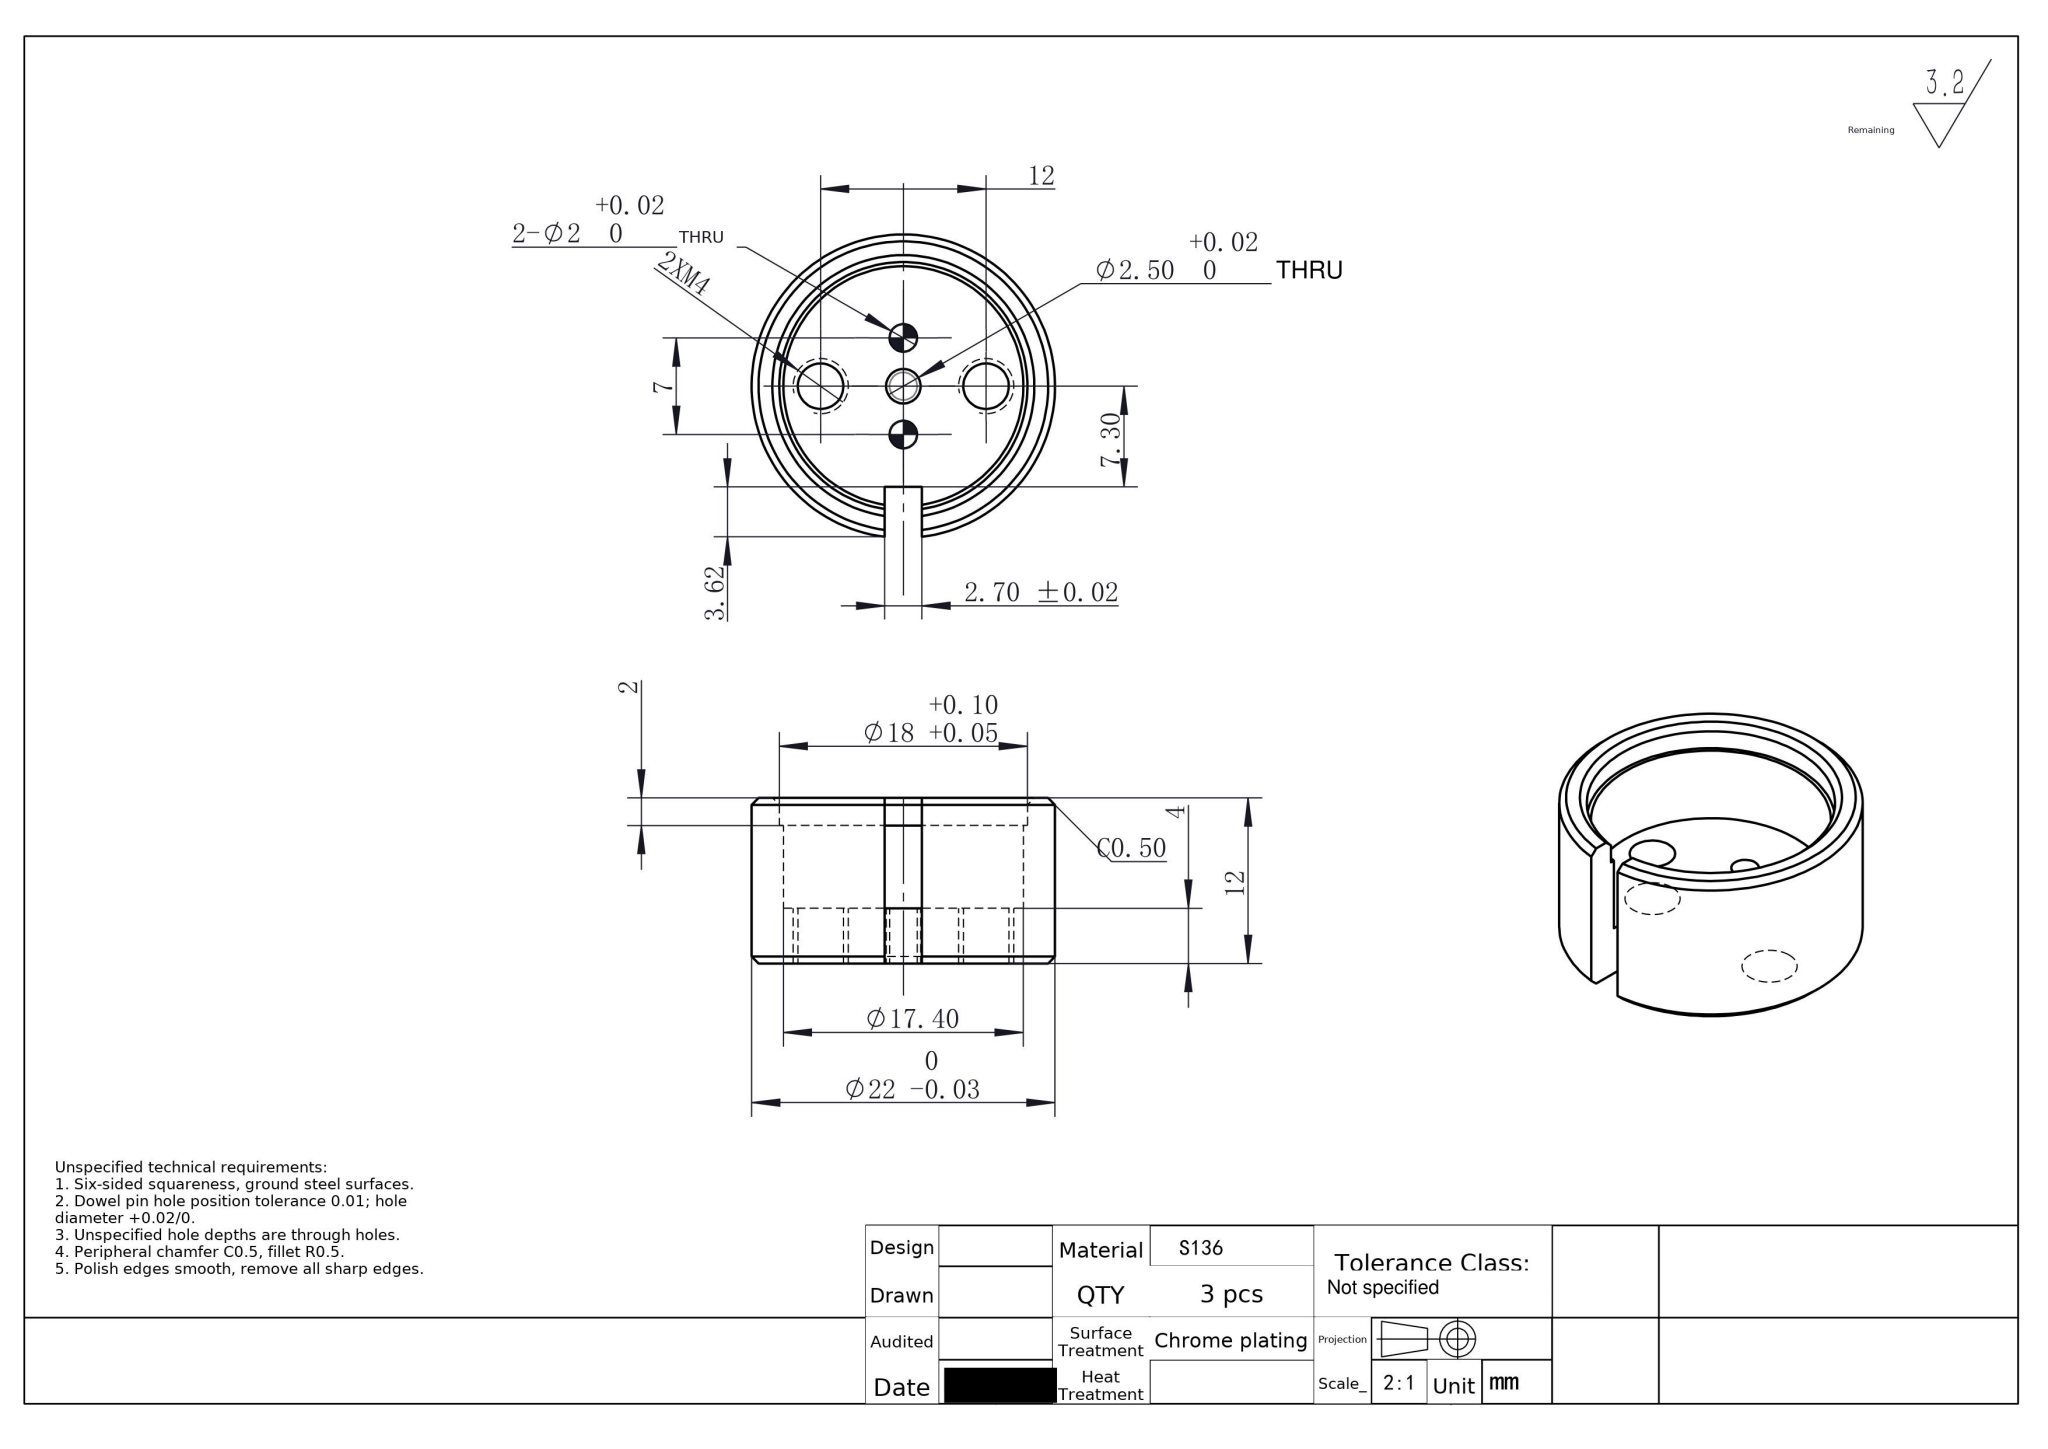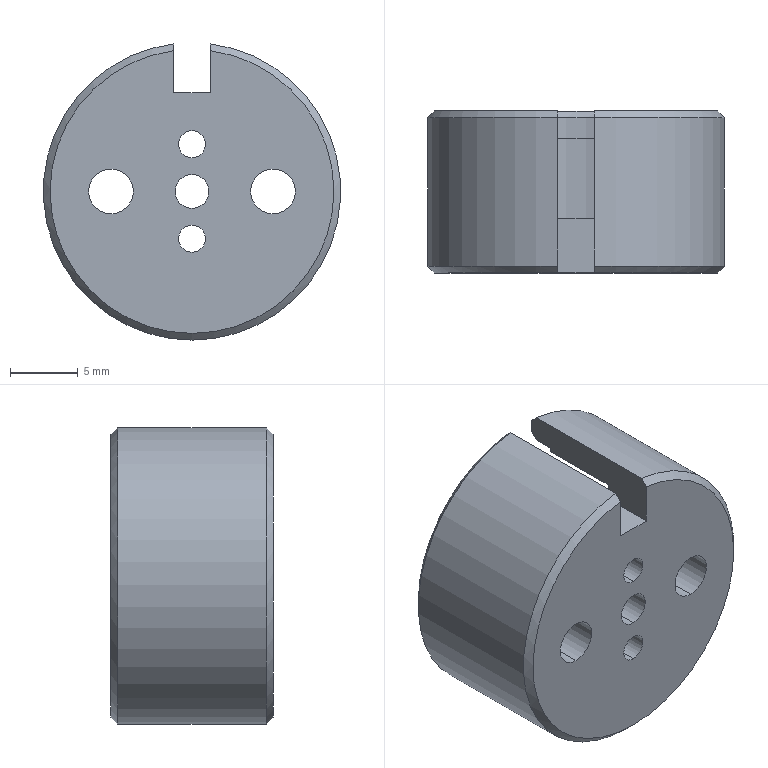Part | NX | mm | 1 solid | 25 faces | box 22 x 12 x 21.92 mm | volume 2402 mm3 | cylinder 14 | plane 7 | cone 4 | commonest cylinder face diameters 2 x4 3.3 x4 22 x2 2.5 x2 18 x1 17.4 x1
STEP:
#1=CARTESIAN_POINT('',(0.,0.,-4.5));
#2=VERTEX_POINT('',#1);
#3=CARTESIAN_POINT('',(0.,0.,-2.5));
#4=VERTEX_POINT('',#3);
#5=CARTESIAN_POINT('',(0.,0.,-3.5));
#6=DIRECTION('',(0.,1.,0.));
#7=DIRECTION('',(0.,0.,1.));
#8=AXIS2_PLACEMENT_3D('',#5,#6,#7);
#9=CIRCLE('',#8,1.);
#10=EDGE_CURVE('',#2,#4,#9,.T.);
#11=ORIENTED_EDGE('',*,*,#10,.F.);
#12=CARTESIAN_POINT('',(0.,4.,-4.5));
#13=VERTEX_POINT('',#12);
#14=CARTESIAN_POINT('',(0.,4.,-4.5));
#15=DIRECTION('',(0.,1.,0.));
#16=VECTOR('',#15,1000.);
#17=LINE('',#14,#16);
#18=EDGE_CURVE('',#2,#13,#17,.T.);
#19=ORIENTED_EDGE('',*,*,#18,.T.);
#20=CARTESIAN_POINT('',(0.,4.,-2.5));
#21=VERTEX_POINT('',#20);
#22=CARTESIAN_POINT('',(0.,4.,-3.5));
#23=DIRECTION('',(0.,1.,0.));
#24=DIRECTION('',(0.,0.,1.));
#25=AXIS2_PLACEMENT_3D('',#22,#23,#24);
#26=CIRCLE('',#25,1.);
#27=EDGE_CURVE('',#13,#21,#26,.T.);
#28=ORIENTED_EDGE('',*,*,#27,.T.);
#29=CARTESIAN_POINT('',(0.,4.,-2.5));
#30=DIRECTION('',(0.,1.,0.));
#31=VECTOR('',#30,1000.);
#32=LINE('',#29,#31);
#33=EDGE_CURVE('',#4,#21,#32,.T.);
#34=ORIENTED_EDGE('',*,*,#33,.F.);
#35=EDGE_LOOP('',(#11,#19,#28,#34));
#36=FACE_OUTER_BOUND('',#35,.T.);
#37=CARTESIAN_POINT('',(0.,4.,-3.5));
#38=DIRECTION('',(0.,1.,0.));
#39=DIRECTION('',(0.,0.,1.));
#40=AXIS2_PLACEMENT_3D('',#37,#38,#39);
#41=CYLINDRICAL_SURFACE('',#40,1.);
#42=ADVANCED_FACE('',(#36),#41,.F.);
#43=CARTESIAN_POINT('',(0.,0.,2.5));
#44=VERTEX_POINT('',#43);
#45=CARTESIAN_POINT('',(0.,0.,4.5));
#46=VERTEX_POINT('',#45);
#47=CARTESIAN_POINT('',(0.,0.,3.5));
#48=DIRECTION('',(0.,1.,0.));
#49=DIRECTION('',(0.,0.,1.));
#50=AXIS2_PLACEMENT_3D('',#47,#48,#49);
#51=CIRCLE('',#50,1.);
#52=EDGE_CURVE('',#44,#46,#51,.T.);
#53=ORIENTED_EDGE('',*,*,#52,.F.);
#54=CARTESIAN_POINT('',(0.,4.,2.5));
#55=VERTEX_POINT('',#54);
#56=CARTESIAN_POINT('',(0.,4.,2.5));
#57=DIRECTION('',(0.,1.,0.));
#58=VECTOR('',#57,1000.);
#59=LINE('',#56,#58);
#60=EDGE_CURVE('',#44,#55,#59,.T.);
#61=ORIENTED_EDGE('',*,*,#60,.T.);
#62=CARTESIAN_POINT('',(0.,4.,4.5));
#63=VERTEX_POINT('',#62);
#64=CARTESIAN_POINT('',(0.,4.,3.5));
#65=DIRECTION('',(0.,1.,0.));
#66=DIRECTION('',(0.,0.,1.));
#67=AXIS2_PLACEMENT_3D('',#64,#65,#66);
#68=CIRCLE('',#67,1.);
#69=EDGE_CURVE('',#55,#63,#68,.T.);
#70=ORIENTED_EDGE('',*,*,#69,.T.);
#71=CARTESIAN_POINT('',(0.,4.,4.5));
#72=DIRECTION('',(0.,1.,0.));
#73=VECTOR('',#72,1000.);
#74=LINE('',#71,#73);
#75=EDGE_CURVE('',#46,#63,#74,.T.);
#76=ORIENTED_EDGE('',*,*,#75,.F.);
#77=EDGE_LOOP('',(#53,#61,#70,#76));
#78=FACE_OUTER_BOUND('',#77,.T.);
#79=CARTESIAN_POINT('',(0.,4.,3.5));
#80=DIRECTION('',(0.,1.,0.));
#81=DIRECTION('',(0.,0.,1.));
#82=AXIS2_PLACEMENT_3D('',#79,#80,#81);
#83=CYLINDRICAL_SURFACE('',#82,1.);
#84=ADVANCED_FACE('',(#78),#83,.F.);
#85=CARTESIAN_POINT('',(0.,12.,-10.5));
#86=VERTEX_POINT('',#85);
#87=CARTESIAN_POINT('',(-1.35,12.,10.413));
#88=VERTEX_POINT('',#87);
#89=CARTESIAN_POINT('',(0.,12.,0.));
#90=DIRECTION('',(0.,1.,0.));
#91=DIRECTION('',(0.,0.,1.));
#92=AXIS2_PLACEMENT_3D('',#89,#90,#91);
#93=CIRCLE('',#92,10.5);
#94=EDGE_CURVE('',#86,#88,#93,.T.);
#95=ORIENTED_EDGE('',*,*,#94,.F.);
#96=CARTESIAN_POINT('',(0.,11.5,-11.));
#97=VERTEX_POINT('',#96);
#98=CARTESIAN_POINT('',(0.,12.,-10.5));
#99=DIRECTION('',(0.,-0.7071,-0.7071));
#100=VECTOR('',#99,1000.);
#101=LINE('',#98,#100);
#102=EDGE_CURVE('',#86,#97,#101,.T.);
#103=ORIENTED_EDGE('',*,*,#102,.T.);
#104=CARTESIAN_POINT('',(-1.35,11.5,10.917));
#105=VERTEX_POINT('',#104);
#106=CARTESIAN_POINT('',(0.,11.5,0.));
#107=DIRECTION('',(0.,-1.,0.));
#108=DIRECTION('',(0.,0.,1.));
#109=AXIS2_PLACEMENT_3D('',#106,#107,#108);
#110=CIRCLE('',#109,11.);
#111=EDGE_CURVE('',#105,#97,#110,.T.);
#112=ORIENTED_EDGE('',*,*,#111,.F.);
#113=CARTESIAN_POINT('',(-1.35,12.,10.413));
#114=CARTESIAN_POINT('',(-1.35,11.833,10.581));
#115=CARTESIAN_POINT('',(-1.35,11.667,10.749));
#116=CARTESIAN_POINT('',(-1.35,11.5,10.917));
#117=B_SPLINE_CURVE_WITH_KNOTS('',3,(#113,#114,#115,#116),.UNSPECIFIED.,.F.,.F.,(4,4),(0.006562,0.007272),.UNSPECIFIED.);
#118=EDGE_CURVE('',#88,#105,#117,.T.);
#119=ORIENTED_EDGE('',*,*,#118,.F.);
#120=EDGE_LOOP('',(#95,#103,#112,#119));
#121=FACE_OUTER_BOUND('',#120,.T.);
#122=CARTESIAN_POINT('',(0.,12.,0.));
#123=DIRECTION('',(0.,-1.,0.));
#124=DIRECTION('',(0.,0.,-1.));
#125=AXIS2_PLACEMENT_3D('',#122,#123,#124);
#126=CONICAL_SURFACE('',#125,10.5,0.7854);
#127=ADVANCED_FACE('',(#121),#126,.T.);
#128=ORIENTED_EDGE('',*,*,#111,.T.);
#129=CARTESIAN_POINT('',(0.,0.5,-11.));
#130=VERTEX_POINT('',#129);
#131=CARTESIAN_POINT('',(0.,12.,-11.));
#132=DIRECTION('',(0.,-1.,0.));
#133=VECTOR('',#132,1000.);
#134=LINE('',#131,#133);
#135=EDGE_CURVE('',#97,#130,#134,.T.);
#136=ORIENTED_EDGE('',*,*,#135,.T.);
#137=CARTESIAN_POINT('',(-1.35,0.5,10.917));
#138=VERTEX_POINT('',#137);
#139=CARTESIAN_POINT('',(0.,0.5,0.));
#140=DIRECTION('',(0.,1.,0.));
#141=DIRECTION('',(0.,0.,1.));
#142=AXIS2_PLACEMENT_3D('',#139,#140,#141);
#143=CIRCLE('',#142,11.);
#144=EDGE_CURVE('',#130,#138,#143,.T.);
#145=ORIENTED_EDGE('',*,*,#144,.T.);
#146=CARTESIAN_POINT('',(-1.35,12.,10.917));
#147=DIRECTION('',(0.,1.,0.));
#148=VECTOR('',#147,1000.);
#149=LINE('',#146,#148);
#150=EDGE_CURVE('',#138,#105,#149,.T.);
#151=ORIENTED_EDGE('',*,*,#150,.T.);
#152=EDGE_LOOP('',(#128,#136,#145,#151));
#153=FACE_OUTER_BOUND('',#152,.T.);
#154=CARTESIAN_POINT('',(0.,12.,0.));
#155=DIRECTION('',(0.,-1.,0.));
#156=DIRECTION('',(0.,0.,-1.));
#157=AXIS2_PLACEMENT_3D('',#154,#155,#156);
#158=CYLINDRICAL_SURFACE('',#157,11.);
#159=ADVANCED_FACE('',(#153),#158,.T.);
#160=CARTESIAN_POINT('',(0.,0.,-1.25));
#161=VERTEX_POINT('',#160);
#162=CARTESIAN_POINT('',(0.,0.,1.25));
#163=VERTEX_POINT('',#162);
#164=CARTESIAN_POINT('',(0.,0.,0.));
#165=DIRECTION('',(0.,1.,0.));
#166=DIRECTION('',(0.,0.,1.));
#167=AXIS2_PLACEMENT_3D('',#164,#165,#166);
#168=CIRCLE('',#167,1.25);
#169=EDGE_CURVE('',#161,#163,#168,.T.);
#170=ORIENTED_EDGE('',*,*,#169,.F.);
#171=CARTESIAN_POINT('',(0.,4.,-1.25));
#172=VERTEX_POINT('',#171);
#173=CARTESIAN_POINT('',(0.,0.,-1.25));
#174=DIRECTION('',(0.,1.,0.));
#175=VECTOR('',#174,1000.);
#176=LINE('',#173,#175);
#177=EDGE_CURVE('',#161,#172,#176,.T.);
#178=ORIENTED_EDGE('',*,*,#177,.T.);
#179=CARTESIAN_POINT('',(0.,4.,1.25));
#180=VERTEX_POINT('',#179);
#181=CARTESIAN_POINT('',(0.,4.,0.));
#182=DIRECTION('',(0.,-1.,0.));
#183=DIRECTION('',(0.,0.,1.));
#184=AXIS2_PLACEMENT_3D('',#181,#182,#183);
#185=CIRCLE('',#184,1.25);
#186=EDGE_CURVE('',#180,#172,#185,.T.);
#187=ORIENTED_EDGE('',*,*,#186,.F.);
#188=CARTESIAN_POINT('',(0.,0.,1.25));
#189=DIRECTION('',(0.,1.,0.));
#190=VECTOR('',#189,1000.);
#191=LINE('',#188,#190);
#192=EDGE_CURVE('',#163,#180,#191,.T.);
#193=ORIENTED_EDGE('',*,*,#192,.F.);
#194=EDGE_LOOP('',(#170,#178,#187,#193));
#195=FACE_OUTER_BOUND('',#194,.T.);
#196=CARTESIAN_POINT('',(0.,0.,0.));
#197=DIRECTION('',(0.,1.,0.));
#198=DIRECTION('',(0.,0.,1.));
#199=AXIS2_PLACEMENT_3D('',#196,#197,#198);
#200=CYLINDRICAL_SURFACE('',#199,1.25);
#201=ADVANCED_FACE('',(#195),#200,.F.);
#202=CARTESIAN_POINT('',(-6.,4.,1.65));
#203=VERTEX_POINT('',#202);
#204=CARTESIAN_POINT('',(-6.,4.,-1.65));
#205=VERTEX_POINT('',#204);
#206=CARTESIAN_POINT('',(-6.,4.,0.));
#207=DIRECTION('',(0.,-1.,0.));
#208=DIRECTION('',(0.,0.,1.));
#209=AXIS2_PLACEMENT_3D('',#206,#207,#208);
#210=CIRCLE('',#209,1.65);
#211=EDGE_CURVE('',#203,#205,#210,.T.);
#212=ORIENTED_EDGE('',*,*,#211,.F.);
#213=CARTESIAN_POINT('',(-6.,-0.,1.65));
#214=VERTEX_POINT('',#213);
#215=CARTESIAN_POINT('',(-6.,0.,1.65));
#216=DIRECTION('',(0.,-1.,0.));
#217=VECTOR('',#216,1000.);
#218=LINE('',#215,#217);
#219=EDGE_CURVE('',#203,#214,#218,.T.);
#220=ORIENTED_EDGE('',*,*,#219,.T.);
#221=CARTESIAN_POINT('',(-6.,-0.,-1.65));
#222=VERTEX_POINT('',#221);
#223=CARTESIAN_POINT('',(-6.,-0.,0.));
#224=DIRECTION('',(0.,-1.,0.));
#225=DIRECTION('',(0.,0.,-1.));
#226=AXIS2_PLACEMENT_3D('',#223,#224,#225);
#227=CIRCLE('',#226,1.65);
#228=EDGE_CURVE('',#214,#222,#227,.T.);
#229=ORIENTED_EDGE('',*,*,#228,.T.);
#230=CARTESIAN_POINT('',(-6.,0.,-1.65));
#231=DIRECTION('',(0.,-1.,0.));
#232=VECTOR('',#231,1000.);
#233=LINE('',#230,#232);
#234=EDGE_CURVE('',#205,#222,#233,.T.);
#235=ORIENTED_EDGE('',*,*,#234,.F.);
#236=EDGE_LOOP('',(#212,#220,#229,#235));
#237=FACE_OUTER_BOUND('',#236,.T.);
#238=CARTESIAN_POINT('',(-6.,0.,0.));
#239=DIRECTION('',(0.,-1.,0.));
#240=DIRECTION('',(0.,0.,-1.));
#241=AXIS2_PLACEMENT_3D('',#238,#239,#240);
#242=CYLINDRICAL_SURFACE('',#241,1.65);
#243=ADVANCED_FACE('',(#237),#242,.F.);
#244=CARTESIAN_POINT('',(6.,4.,1.65));
#245=VERTEX_POINT('',#244);
#246=CARTESIAN_POINT('',(6.,4.,-1.65));
#247=VERTEX_POINT('',#246);
#248=CARTESIAN_POINT('',(6.,4.,0.));
#249=DIRECTION('',(0.,-1.,0.));
#250=DIRECTION('',(0.,0.,1.));
#251=AXIS2_PLACEMENT_3D('',#248,#249,#250);
#252=CIRCLE('',#251,1.65);
#253=EDGE_CURVE('',#245,#247,#252,.T.);
#254=ORIENTED_EDGE('',*,*,#253,.F.);
#255=CARTESIAN_POINT('',(6.,-0.,1.65));
#256=VERTEX_POINT('',#255);
#257=CARTESIAN_POINT('',(6.,0.,1.65));
#258=DIRECTION('',(0.,-1.,0.));
#259=VECTOR('',#258,1000.);
#260=LINE('',#257,#259);
#261=EDGE_CURVE('',#245,#256,#260,.T.);
#262=ORIENTED_EDGE('',*,*,#261,.T.);
#263=CARTESIAN_POINT('',(6.,-0.,-1.65));
#264=VERTEX_POINT('',#263);
#265=CARTESIAN_POINT('',(6.,-0.,0.));
#266=DIRECTION('',(0.,-1.,0.));
#267=DIRECTION('',(0.,0.,-1.));
#268=AXIS2_PLACEMENT_3D('',#265,#266,#267);
#269=CIRCLE('',#268,1.65);
#270=EDGE_CURVE('',#256,#264,#269,.T.);
#271=ORIENTED_EDGE('',*,*,#270,.T.);
#272=CARTESIAN_POINT('',(6.,0.,-1.65));
#273=DIRECTION('',(0.,-1.,0.));
#274=VECTOR('',#273,1000.);
#275=LINE('',#272,#274);
#276=EDGE_CURVE('',#247,#264,#275,.T.);
#277=ORIENTED_EDGE('',*,*,#276,.F.);
#278=EDGE_LOOP('',(#254,#262,#271,#277));
#279=FACE_OUTER_BOUND('',#278,.T.);
#280=CARTESIAN_POINT('',(6.,0.,0.));
#281=DIRECTION('',(0.,-1.,0.));
#282=DIRECTION('',(0.,0.,-1.));
#283=AXIS2_PLACEMENT_3D('',#280,#281,#282);
#284=CYLINDRICAL_SURFACE('',#283,1.65);
#285=ADVANCED_FACE('',(#279),#284,.F.);
#286=ORIENTED_EDGE('',*,*,#261,.F.);
#287=CARTESIAN_POINT('',(6.,4.,0.));
#288=DIRECTION('',(0.,-1.,0.));
#289=DIRECTION('',(0.,0.,1.));
#290=AXIS2_PLACEMENT_3D('',#287,#288,#289);
#291=CIRCLE('',#290,1.65);
#292=EDGE_CURVE('',#247,#245,#291,.T.);
#293=ORIENTED_EDGE('',*,*,#292,.F.);
#294=ORIENTED_EDGE('',*,*,#276,.T.);
#295=CARTESIAN_POINT('',(6.,-0.,0.));
#296=DIRECTION('',(0.,-1.,0.));
#297=DIRECTION('',(0.,0.,-1.));
#298=AXIS2_PLACEMENT_3D('',#295,#296,#297);
#299=CIRCLE('',#298,1.65);
#300=EDGE_CURVE('',#264,#256,#299,.T.);
#301=ORIENTED_EDGE('',*,*,#300,.T.);
#302=EDGE_LOOP('',(#286,#293,#294,#301));
#303=FACE_OUTER_BOUND('',#302,.T.);
#304=CARTESIAN_POINT('',(6.,0.,0.));
#305=DIRECTION('',(0.,-1.,0.));
#306=DIRECTION('',(0.,0.,-1.));
#307=AXIS2_PLACEMENT_3D('',#304,#305,#306);
#308=CYLINDRICAL_SURFACE('',#307,1.65);
#309=ADVANCED_FACE('',(#303),#308,.F.);
#310=ORIENTED_EDGE('',*,*,#219,.F.);
#311=CARTESIAN_POINT('',(-6.,4.,0.));
#312=DIRECTION('',(0.,-1.,0.));
#313=DIRECTION('',(0.,0.,1.));
#314=AXIS2_PLACEMENT_3D('',#311,#312,#313);
#315=CIRCLE('',#314,1.65);
#316=EDGE_CURVE('',#205,#203,#315,.T.);
#317=ORIENTED_EDGE('',*,*,#316,.F.);
#318=ORIENTED_EDGE('',*,*,#234,.T.);
#319=CARTESIAN_POINT('',(-6.,-0.,0.));
#320=DIRECTION('',(0.,-1.,0.));
#321=DIRECTION('',(0.,0.,-1.));
#322=AXIS2_PLACEMENT_3D('',#319,#320,#321);
#323=CIRCLE('',#322,1.65);
#324=EDGE_CURVE('',#222,#214,#323,.T.);
#325=ORIENTED_EDGE('',*,*,#324,.T.);
#326=EDGE_LOOP('',(#310,#317,#318,#325));
#327=FACE_OUTER_BOUND('',#326,.T.);
#328=CARTESIAN_POINT('',(-6.,0.,0.));
#329=DIRECTION('',(0.,-1.,0.));
#330=DIRECTION('',(0.,0.,-1.));
#331=AXIS2_PLACEMENT_3D('',#328,#329,#330);
#332=CYLINDRICAL_SURFACE('',#331,1.65);
#333=ADVANCED_FACE('',(#327),#332,.F.);
#334=ORIENTED_EDGE('',*,*,#177,.F.);
#335=CARTESIAN_POINT('',(0.,0.,0.));
#336=DIRECTION('',(0.,1.,0.));
#337=DIRECTION('',(0.,0.,1.));
#338=AXIS2_PLACEMENT_3D('',#335,#336,#337);
#339=CIRCLE('',#338,1.25);
#340=EDGE_CURVE('',#163,#161,#339,.T.);
#341=ORIENTED_EDGE('',*,*,#340,.F.);
#342=ORIENTED_EDGE('',*,*,#192,.T.);
#343=CARTESIAN_POINT('',(0.,4.,0.));
#344=DIRECTION('',(0.,-1.,0.));
#345=DIRECTION('',(0.,0.,1.));
#346=AXIS2_PLACEMENT_3D('',#343,#344,#345);
#347=CIRCLE('',#346,1.25);
#348=EDGE_CURVE('',#172,#180,#347,.T.);
#349=ORIENTED_EDGE('',*,*,#348,.F.);
#350=EDGE_LOOP('',(#334,#341,#342,#349));
#351=FACE_OUTER_BOUND('',#350,.T.);
#352=CARTESIAN_POINT('',(0.,0.,0.));
#353=DIRECTION('',(0.,1.,0.));
#354=DIRECTION('',(0.,0.,1.));
#355=AXIS2_PLACEMENT_3D('',#352,#353,#354);
#356=CYLINDRICAL_SURFACE('',#355,1.25);
#357=ADVANCED_FACE('',(#351),#356,.F.);
#358=ORIENTED_EDGE('',*,*,#135,.F.);
#359=CARTESIAN_POINT('',(1.35,11.5,10.917));
#360=VERTEX_POINT('',#359);
#361=CARTESIAN_POINT('',(0.,11.5,0.));
#362=DIRECTION('',(0.,-1.,0.));
#363=DIRECTION('',(0.,0.,1.));
#364=AXIS2_PLACEMENT_3D('',#361,#362,#363);
#365=CIRCLE('',#364,11.);
#366=EDGE_CURVE('',#97,#360,#365,.T.);
#367=ORIENTED_EDGE('',*,*,#366,.T.);
#368=CARTESIAN_POINT('',(1.35,0.5,10.917));
#369=VERTEX_POINT('',#368);
#370=CARTESIAN_POINT('',(1.35,12.,10.917));
#371=DIRECTION('',(0.,-1.,0.));
#372=VECTOR('',#371,1000.);
#373=LINE('',#370,#372);
#374=EDGE_CURVE('',#360,#369,#373,.T.);
#375=ORIENTED_EDGE('',*,*,#374,.T.);
#376=CARTESIAN_POINT('',(0.,0.5,0.));
#377=DIRECTION('',(0.,1.,0.));
#378=DIRECTION('',(0.,0.,1.));
#379=AXIS2_PLACEMENT_3D('',#376,#377,#378);
#380=CIRCLE('',#379,11.);
#381=EDGE_CURVE('',#369,#130,#380,.T.);
#382=ORIENTED_EDGE('',*,*,#381,.T.);
#383=EDGE_LOOP('',(#358,#367,#375,#382));
#384=FACE_OUTER_BOUND('',#383,.T.);
#385=CARTESIAN_POINT('',(0.,12.,0.));
#386=DIRECTION('',(0.,-1.,0.));
#387=DIRECTION('',(0.,0.,-1.));
#388=AXIS2_PLACEMENT_3D('',#385,#386,#387);
#389=CYLINDRICAL_SURFACE('',#388,11.);
#390=ADVANCED_FACE('',(#384),#389,.T.);
#391=CARTESIAN_POINT('',(-1.35,12.,9.404));
#392=VERTEX_POINT('',#391);
#393=CARTESIAN_POINT('',(-1.35,12.,7.3));
#394=DIRECTION('',(0.,0.,1.));
#395=VECTOR('',#394,1000.);
#396=LINE('',#393,#395);
#397=EDGE_CURVE('',#392,#88,#396,.T.);
#398=ORIENTED_EDGE('',*,*,#397,.F.);
#399=CARTESIAN_POINT('',(1.35,12.,9.404));
#400=VERTEX_POINT('',#399);
#401=CARTESIAN_POINT('',(0.,12.,0.));
#402=DIRECTION('',(0.,-1.,0.));
#403=DIRECTION('',(0.,0.,1.));
#404=AXIS2_PLACEMENT_3D('',#401,#402,#403);
#405=CIRCLE('',#404,9.5);
#406=EDGE_CURVE('',#392,#400,#405,.T.);
#407=ORIENTED_EDGE('',*,*,#406,.T.);
#408=CARTESIAN_POINT('',(1.35,12.,10.413));
#409=VERTEX_POINT('',#408);
#410=CARTESIAN_POINT('',(1.35,12.,7.3));
#411=DIRECTION('',(-0.,0.,-1.));
#412=VECTOR('',#411,1000.);
#413=LINE('',#410,#412);
#414=EDGE_CURVE('',#409,#400,#413,.T.);
#415=ORIENTED_EDGE('',*,*,#414,.F.);
#416=CARTESIAN_POINT('',(0.,12.,0.));
#417=DIRECTION('',(0.,1.,0.));
#418=DIRECTION('',(0.,0.,1.));
#419=AXIS2_PLACEMENT_3D('',#416,#417,#418);
#420=CIRCLE('',#419,10.5);
#421=EDGE_CURVE('',#409,#86,#420,.T.);
#422=ORIENTED_EDGE('',*,*,#421,.T.);
#423=ORIENTED_EDGE('',*,*,#94,.T.);
#424=EDGE_LOOP('',(#398,#407,#415,#422,#423));
#425=FACE_OUTER_BOUND('',#424,.T.);
#426=CARTESIAN_POINT('',(0.,12.,0.));
#427=DIRECTION('',(0.,1.,0.));
#428=DIRECTION('',(0.,0.,1.));
#429=AXIS2_PLACEMENT_3D('',#426,#427,#428);
#430=PLANE('',#429);
#431=ADVANCED_FACE('',(#425),#430,.T.);
#432=CARTESIAN_POINT('',(0.,0.,-3.5));
#433=DIRECTION('',(0.,1.,0.));
#434=DIRECTION('',(0.,0.,1.));
#435=AXIS2_PLACEMENT_3D('',#432,#433,#434);
#436=CIRCLE('',#435,1.);
#437=EDGE_CURVE('',#4,#2,#436,.T.);
#438=ORIENTED_EDGE('',*,*,#437,.T.);
#439=ORIENTED_EDGE('',*,*,#10,.T.);
#440=EDGE_LOOP('',(#438,#439));
#441=FACE_BOUND('',#440,.T.);
#442=CARTESIAN_POINT('',(0.,0.,3.5));
#443=DIRECTION('',(0.,1.,0.));
#444=DIRECTION('',(0.,0.,1.));
#445=AXIS2_PLACEMENT_3D('',#442,#443,#444);
#446=CIRCLE('',#445,1.);
#447=EDGE_CURVE('',#46,#44,#446,.T.);
#448=ORIENTED_EDGE('',*,*,#447,.T.);
#449=ORIENTED_EDGE('',*,*,#52,.T.);
#450=EDGE_LOOP('',(#448,#449));
#451=FACE_BOUND('',#450,.T.);
#452=ORIENTED_EDGE('',*,*,#340,.T.);
#453=ORIENTED_EDGE('',*,*,#169,.T.);
#454=EDGE_LOOP('',(#452,#453));
#455=FACE_BOUND('',#454,.T.);
#456=CARTESIAN_POINT('',(1.35,0.,7.3));
#457=VERTEX_POINT('',#456);
#458=CARTESIAN_POINT('',(-1.35,0.,7.3));
#459=VERTEX_POINT('',#458);
#460=CARTESIAN_POINT('',(-1.35,0.,7.3));
#461=DIRECTION('',(-1.,0.,0.));
#462=VECTOR('',#461,1000.);
#463=LINE('',#460,#462);
#464=EDGE_CURVE('',#457,#459,#463,.T.);
#465=ORIENTED_EDGE('',*,*,#464,.T.);
#466=CARTESIAN_POINT('',(-1.35,0.,10.413));
#467=VERTEX_POINT('',#466);
#468=CARTESIAN_POINT('',(-1.35,0.,7.3));
#469=DIRECTION('',(0.,0.,1.));
#470=VECTOR('',#469,1000.);
#471=LINE('',#468,#470);
#472=EDGE_CURVE('',#459,#467,#471,.T.);
#473=ORIENTED_EDGE('',*,*,#472,.T.);
#474=CARTESIAN_POINT('',(1.35,0.,10.413));
#475=VERTEX_POINT('',#474);
#476=CARTESIAN_POINT('',(0.,0.,0.));
#477=DIRECTION('',(0.,-1.,0.));
#478=DIRECTION('',(0.,0.,1.));
#479=AXIS2_PLACEMENT_3D('',#476,#477,#478);
#480=CIRCLE('',#479,10.5);
#481=EDGE_CURVE('',#467,#475,#480,.T.);
#482=ORIENTED_EDGE('',*,*,#481,.T.);
#483=CARTESIAN_POINT('',(1.35,0.,7.3));
#484=DIRECTION('',(-0.,0.,-1.));
#485=VECTOR('',#484,1000.);
#486=LINE('',#483,#485);
#487=EDGE_CURVE('',#475,#457,#486,.T.);
#488=ORIENTED_EDGE('',*,*,#487,.T.);
#489=EDGE_LOOP('',(#465,#473,#482,#488));
#490=FACE_OUTER_BOUND('',#489,.T.);
#491=ORIENTED_EDGE('',*,*,#324,.F.);
#492=ORIENTED_EDGE('',*,*,#228,.F.);
#493=EDGE_LOOP('',(#491,#492));
#494=FACE_BOUND('',#493,.T.);
#495=ORIENTED_EDGE('',*,*,#300,.F.);
#496=ORIENTED_EDGE('',*,*,#270,.F.);
#497=EDGE_LOOP('',(#495,#496));
#498=FACE_BOUND('',#497,.T.);
#499=CARTESIAN_POINT('',(0.,0.,0.));
#500=DIRECTION('',(0.,1.,0.));
#501=DIRECTION('',(0.,0.,1.));
#502=AXIS2_PLACEMENT_3D('',#499,#500,#501);
#503=PLANE('',#502);
#504=ADVANCED_FACE('',(#441,#451,#455,#490,#494,#498),#503,.F.);
#505=CARTESIAN_POINT('',(1.35,11.5,8.898));
#506=VERTEX_POINT('',#505);
#507=CARTESIAN_POINT('',(-1.35,11.5,8.898));
#508=VERTEX_POINT('',#507);
#509=CARTESIAN_POINT('',(0.,11.5,0.));
#510=DIRECTION('',(0.,1.,0.));
#511=DIRECTION('',(0.,0.,1.));
#512=AXIS2_PLACEMENT_3D('',#509,#510,#511);
#513=CIRCLE('',#512,9.);
#514=EDGE_CURVE('',#506,#508,#513,.T.);
#515=ORIENTED_EDGE('',*,*,#514,.T.);
#516=CARTESIAN_POINT('',(-1.35,10.,8.898));
#517=VERTEX_POINT('',#516);
#518=CARTESIAN_POINT('',(-1.35,10.,8.898));
#519=DIRECTION('',(0.,-1.,0.));
#520=VECTOR('',#519,1000.);
#521=LINE('',#518,#520);
#522=EDGE_CURVE('',#508,#517,#521,.T.);
#523=ORIENTED_EDGE('',*,*,#522,.T.);
#524=CARTESIAN_POINT('',(1.35,10.,8.898));
#525=VERTEX_POINT('',#524);
#526=CARTESIAN_POINT('',(0.,10.,0.));
#527=DIRECTION('',(0.,1.,0.));
#528=DIRECTION('',(0.,0.,1.));
#529=AXIS2_PLACEMENT_3D('',#526,#527,#528);
#530=CIRCLE('',#529,9.);
#531=EDGE_CURVE('',#525,#517,#530,.T.);
#532=ORIENTED_EDGE('',*,*,#531,.F.);
#533=CARTESIAN_POINT('',(1.35,10.,8.898));
#534=DIRECTION('',(0.,1.,0.));
#535=VECTOR('',#534,1000.);
#536=LINE('',#533,#535);
#537=EDGE_CURVE('',#525,#506,#536,.T.);
#538=ORIENTED_EDGE('',*,*,#537,.T.);
#539=EDGE_LOOP('',(#515,#523,#532,#538));
#540=FACE_OUTER_BOUND('',#539,.T.);
#541=CARTESIAN_POINT('',(0.,10.,0.));
#542=DIRECTION('',(0.,1.,0.));
#543=DIRECTION('',(0.,0.,1.));
#544=AXIS2_PLACEMENT_3D('',#541,#542,#543);
#545=CYLINDRICAL_SURFACE('',#544,9.);
#546=ADVANCED_FACE('',(#540),#545,.F.);
#547=CARTESIAN_POINT('',(-1.35,10.,8.595));
#548=VERTEX_POINT('',#547);
#549=CARTESIAN_POINT('',(-1.35,10.,0.));
#550=DIRECTION('',(0.,0.,1.));
#551=VECTOR('',#550,1000.);
#552=LINE('',#549,#551);
#553=EDGE_CURVE('',#548,#517,#552,.T.);
#554=ORIENTED_EDGE('',*,*,#553,.F.);
#555=CARTESIAN_POINT('',(1.35,10.,8.595));
#556=VERTEX_POINT('',#555);
#557=CARTESIAN_POINT('',(0.,10.,0.));
#558=DIRECTION('',(0.,1.,0.));
#559=DIRECTION('',(0.,0.,1.));
#560=AXIS2_PLACEMENT_3D('',#557,#558,#559);
#561=CIRCLE('',#560,8.7);
#562=EDGE_CURVE('',#556,#548,#561,.T.);
#563=ORIENTED_EDGE('',*,*,#562,.F.);
#564=CARTESIAN_POINT('',(1.35,10.,-0.));
#565=DIRECTION('',(-0.,0.,-1.));
#566=VECTOR('',#565,1000.);
#567=LINE('',#564,#566);
#568=EDGE_CURVE('',#525,#556,#567,.T.);
#569=ORIENTED_EDGE('',*,*,#568,.F.);
#570=ORIENTED_EDGE('',*,*,#531,.T.);
#571=EDGE_LOOP('',(#554,#563,#569,#570));
#572=FACE_OUTER_BOUND('',#571,.T.);
#573=CARTESIAN_POINT('',(0.,10.,0.));
#574=DIRECTION('',(0.,1.,0.));
#575=DIRECTION('',(0.,0.,1.));
#576=AXIS2_PLACEMENT_3D('',#573,#574,#575);
#577=PLANE('',#576);
#578=ADVANCED_FACE('',(#572),#577,.T.);
#579=CARTESIAN_POINT('',(-1.35,0.5,10.917));
#580=CARTESIAN_POINT('',(-1.35,0.3333,10.749));
#581=CARTESIAN_POINT('',(-1.35,0.1666,10.581));
#582=CARTESIAN_POINT('',(-1.35,0.,10.413));
#583=B_SPLINE_CURVE_WITH_KNOTS('',3,(#579,#580,#581,#582),.UNSPECIFIED.,.F.,.F.,(4,4),(0.006381,0.007091),.UNSPECIFIED.);
#584=EDGE_CURVE('',#138,#467,#583,.T.);
#585=ORIENTED_EDGE('',*,*,#584,.F.);
#586=ORIENTED_EDGE('',*,*,#144,.F.);
#587=ORIENTED_EDGE('',*,*,#381,.F.);
#588=CARTESIAN_POINT('',(1.35,0.,10.413));
#589=CARTESIAN_POINT('',(1.35,0.1666,10.581));
#590=CARTESIAN_POINT('',(1.35,0.3333,10.749));
#591=CARTESIAN_POINT('',(1.35,0.5,10.917));
#592=B_SPLINE_CURVE_WITH_KNOTS('',3,(#588,#589,#590,#591),.UNSPECIFIED.,.F.,.F.,(4,4),(0.006562,0.007272),.UNSPECIFIED.);
#593=EDGE_CURVE('',#475,#369,#592,.T.);
#594=ORIENTED_EDGE('',*,*,#593,.F.);
#595=ORIENTED_EDGE('',*,*,#481,.F.);
#596=EDGE_LOOP('',(#585,#586,#587,#594,#595));
#597=FACE_OUTER_BOUND('',#596,.T.);
#598=CARTESIAN_POINT('',(0.,0.5,0.));
#599=DIRECTION('',(0.,1.,0.));
#600=DIRECTION('',(0.,0.,1.));
#601=AXIS2_PLACEMENT_3D('',#598,#599,#600);
#602=CONICAL_SURFACE('',#601,11.,0.7854);
#603=ADVANCED_FACE('',(#597),#602,.T.);
#604=ORIENTED_EDGE('',*,*,#102,.F.);
#605=ORIENTED_EDGE('',*,*,#421,.F.);
#606=CARTESIAN_POINT('',(1.35,11.5,10.917));
#607=CARTESIAN_POINT('',(1.35,11.667,10.749));
#608=CARTESIAN_POINT('',(1.35,11.833,10.581));
#609=CARTESIAN_POINT('',(1.35,12.,10.413));
#610=B_SPLINE_CURVE_WITH_KNOTS('',3,(#606,#607,#608,#609),.UNSPECIFIED.,.F.,.F.,(4,4),(0.006381,0.007091),.UNSPECIFIED.);
#611=EDGE_CURVE('',#360,#409,#610,.T.);
#612=ORIENTED_EDGE('',*,*,#611,.F.);
#613=ORIENTED_EDGE('',*,*,#366,.F.);
#614=EDGE_LOOP('',(#604,#605,#612,#613));
#615=FACE_OUTER_BOUND('',#614,.T.);
#616=CARTESIAN_POINT('',(0.,12.,0.));
#617=DIRECTION('',(0.,-1.,0.));
#618=DIRECTION('',(0.,0.,-1.));
#619=AXIS2_PLACEMENT_3D('',#616,#617,#618);
#620=CONICAL_SURFACE('',#619,10.5,0.7854);
#621=ADVANCED_FACE('',(#615),#620,.T.);
#622=CARTESIAN_POINT('',(-1.35,11.5,8.898));
#623=CARTESIAN_POINT('',(-1.35,11.667,9.067));
#624=CARTESIAN_POINT('',(-1.35,11.833,9.235));
#625=CARTESIAN_POINT('',(-1.35,12.,9.404));
#626=B_SPLINE_CURVE_WITH_KNOTS('',3,(#622,#623,#624,#625),.UNSPECIFIED.,.F.,.F.,(4,4),(0.004218,0.004929),.UNSPECIFIED.);
#627=EDGE_CURVE('',#508,#392,#626,.T.);
#628=ORIENTED_EDGE('',*,*,#627,.F.);
#629=ORIENTED_EDGE('',*,*,#514,.F.);
#630=CARTESIAN_POINT('',(1.35,12.,9.404));
#631=CARTESIAN_POINT('',(1.35,11.833,9.235));
#632=CARTESIAN_POINT('',(1.35,11.667,9.067));
#633=CARTESIAN_POINT('',(1.35,11.5,8.898));
#634=B_SPLINE_CURVE_WITH_KNOTS('',3,(#630,#631,#632,#633),.UNSPECIFIED.,.F.,.F.,(4,4),(0.003541,0.004252),.UNSPECIFIED.);
#635=EDGE_CURVE('',#400,#506,#634,.T.);
#636=ORIENTED_EDGE('',*,*,#635,.F.);
#637=ORIENTED_EDGE('',*,*,#406,.F.);
#638=EDGE_LOOP('',(#628,#629,#636,#637));
#639=FACE_OUTER_BOUND('',#638,.T.);
#640=CARTESIAN_POINT('',(0.,11.5,0.));
#641=DIRECTION('',(0.,1.,0.));
#642=DIRECTION('',(0.,0.,1.));
#643=AXIS2_PLACEMENT_3D('',#640,#641,#642);
#644=CONICAL_SURFACE('',#643,9.,0.7854);
#645=ADVANCED_FACE('',(#639),#644,.F.);
#646=CARTESIAN_POINT('',(0.,4.,-3.5));
#647=DIRECTION('',(0.,1.,0.));
#648=DIRECTION('',(0.,0.,1.));
#649=AXIS2_PLACEMENT_3D('',#646,#647,#648);
#650=CIRCLE('',#649,1.);
#651=EDGE_CURVE('',#21,#13,#650,.T.);
#652=ORIENTED_EDGE('',*,*,#651,.F.);
#653=ORIENTED_EDGE('',*,*,#27,.F.);
#654=EDGE_LOOP('',(#652,#653));
#655=FACE_BOUND('',#654,.T.);
#656=CARTESIAN_POINT('',(0.,4.,3.5));
#657=DIRECTION('',(0.,1.,0.));
#658=DIRECTION('',(0.,0.,1.));
#659=AXIS2_PLACEMENT_3D('',#656,#657,#658);
#660=CIRCLE('',#659,1.);
#661=EDGE_CURVE('',#63,#55,#660,.T.);
#662=ORIENTED_EDGE('',*,*,#661,.F.);
#663=ORIENTED_EDGE('',*,*,#69,.F.);
#664=EDGE_LOOP('',(#662,#663));
#665=FACE_BOUND('',#664,.T.);
#666=CARTESIAN_POINT('',(-1.35,4.,7.3));
#667=VERTEX_POINT('',#666);
#668=CARTESIAN_POINT('',(-1.35,4.,8.595));
#669=VERTEX_POINT('',#668);
#670=CARTESIAN_POINT('',(-1.35,4.,0.));
#671=DIRECTION('',(0.,0.,1.));
#672=VECTOR('',#671,1000.);
#673=LINE('',#670,#672);
#674=EDGE_CURVE('',#667,#669,#673,.T.);
#675=ORIENTED_EDGE('',*,*,#674,.F.);
#676=CARTESIAN_POINT('',(1.35,4.,7.3));
#677=VERTEX_POINT('',#676);
#678=CARTESIAN_POINT('',(0.,4.,7.3));
#679=DIRECTION('',(-1.,0.,0.));
#680=VECTOR('',#679,1000.);
#681=LINE('',#678,#680);
#682=EDGE_CURVE('',#677,#667,#681,.T.);
#683=ORIENTED_EDGE('',*,*,#682,.F.);
#684=CARTESIAN_POINT('',(1.35,4.,8.595));
#685=VERTEX_POINT('',#684);
#686=CARTESIAN_POINT('',(1.35,4.,-0.));
#687=DIRECTION('',(-0.,0.,-1.));
#688=VECTOR('',#687,1000.);
#689=LINE('',#686,#688);
#690=EDGE_CURVE('',#685,#677,#689,.T.);
#691=ORIENTED_EDGE('',*,*,#690,.F.);
#692=CARTESIAN_POINT('',(0.,4.,0.));
#693=DIRECTION('',(0.,1.,0.));
#694=DIRECTION('',(0.,0.,1.));
#695=AXIS2_PLACEMENT_3D('',#692,#693,#694);
#696=CIRCLE('',#695,8.7);
#697=EDGE_CURVE('',#685,#669,#696,.T.);
#698=ORIENTED_EDGE('',*,*,#697,.T.);
#699=EDGE_LOOP('',(#675,#683,#691,#698));
#700=FACE_OUTER_BOUND('',#699,.T.);
#701=ORIENTED_EDGE('',*,*,#186,.T.);
#702=ORIENTED_EDGE('',*,*,#348,.T.);
#703=EDGE_LOOP('',(#701,#702));
#704=FACE_BOUND('',#703,.T.);
#705=ORIENTED_EDGE('',*,*,#316,.T.);
#706=ORIENTED_EDGE('',*,*,#211,.T.);
#707=EDGE_LOOP('',(#705,#706));
#708=FACE_BOUND('',#707,.T.);
#709=ORIENTED_EDGE('',*,*,#292,.T.);
#710=ORIENTED_EDGE('',*,*,#253,.T.);
#711=EDGE_LOOP('',(#709,#710));
#712=FACE_BOUND('',#711,.T.);
#713=CARTESIAN_POINT('',(0.,4.,0.));
#714=DIRECTION('',(0.,1.,0.));
#715=DIRECTION('',(0.,0.,1.));
#716=AXIS2_PLACEMENT_3D('',#713,#714,#715);
#717=PLANE('',#716);
#718=ADVANCED_FACE('',(#655,#665,#700,#704,#708,#712),#717,.T.);
#719=ORIENTED_EDGE('',*,*,#562,.T.);
#720=CARTESIAN_POINT('',(-1.35,4.,8.595));
#721=DIRECTION('',(0.,-1.,0.));
#722=VECTOR('',#721,1000.);
#723=LINE('',#720,#722);
#724=EDGE_CURVE('',#548,#669,#723,.T.);
#725=ORIENTED_EDGE('',*,*,#724,.T.);
#726=ORIENTED_EDGE('',*,*,#697,.F.);
#727=CARTESIAN_POINT('',(1.35,4.,8.595));
#728=DIRECTION('',(0.,1.,0.));
#729=VECTOR('',#728,1000.);
#730=LINE('',#727,#729);
#731=EDGE_CURVE('',#685,#556,#730,.T.);
#732=ORIENTED_EDGE('',*,*,#731,.T.);
#733=EDGE_LOOP('',(#719,#725,#726,#732));
#734=FACE_OUTER_BOUND('',#733,.T.);
#735=CARTESIAN_POINT('',(0.,4.,0.));
#736=DIRECTION('',(0.,1.,0.));
#737=DIRECTION('',(0.,0.,1.));
#738=AXIS2_PLACEMENT_3D('',#735,#736,#737);
#739=CYLINDRICAL_SURFACE('',#738,8.7);
#740=ADVANCED_FACE('',(#734),#739,.F.);
#741=ORIENTED_EDGE('',*,*,#584,.T.);
#742=ORIENTED_EDGE('',*,*,#472,.F.);
#743=CARTESIAN_POINT('',(-1.35,0.,7.3));
#744=DIRECTION('',(0.,1.,0.));
#745=VECTOR('',#744,1000.);
#746=LINE('',#743,#745);
#747=EDGE_CURVE('',#459,#667,#746,.T.);
#748=ORIENTED_EDGE('',*,*,#747,.T.);
#749=ORIENTED_EDGE('',*,*,#674,.T.);
#750=ORIENTED_EDGE('',*,*,#724,.F.);
#751=ORIENTED_EDGE('',*,*,#553,.T.);
#752=ORIENTED_EDGE('',*,*,#522,.F.);
#753=ORIENTED_EDGE('',*,*,#627,.T.);
#754=ORIENTED_EDGE('',*,*,#397,.T.);
#755=ORIENTED_EDGE('',*,*,#118,.T.);
#756=ORIENTED_EDGE('',*,*,#150,.F.);
#757=EDGE_LOOP('',(#741,#742,#748,#749,#750,#751,#752,#753,#754,#755,#756));
#758=FACE_OUTER_BOUND('',#757,.T.);
#759=CARTESIAN_POINT('',(-1.35,0.,7.3));
#760=DIRECTION('',(-1.,0.,0.));
#761=DIRECTION('',(0.,0.,1.));
#762=AXIS2_PLACEMENT_3D('',#759,#760,#761);
#763=PLANE('',#762);
#764=ADVANCED_FACE('',(#758),#763,.F.);
#765=ORIENTED_EDGE('',*,*,#682,.T.);
#766=ORIENTED_EDGE('',*,*,#747,.F.);
#767=ORIENTED_EDGE('',*,*,#464,.F.);
#768=CARTESIAN_POINT('',(1.35,0.,7.3));
#769=DIRECTION('',(0.,1.,0.));
#770=VECTOR('',#769,1000.);
#771=LINE('',#768,#770);
#772=EDGE_CURVE('',#457,#677,#771,.T.);
#773=ORIENTED_EDGE('',*,*,#772,.T.);
#774=EDGE_LOOP('',(#765,#766,#767,#773));
#775=FACE_OUTER_BOUND('',#774,.T.);
#776=CARTESIAN_POINT('',(-1.35,0.,7.3));
#777=DIRECTION('',(0.,0.,-1.));
#778=DIRECTION('',(-1.,0.,0.));
#779=AXIS2_PLACEMENT_3D('',#776,#777,#778);
#780=PLANE('',#779);
#781=ADVANCED_FACE('',(#775),#780,.F.);
#782=ORIENTED_EDGE('',*,*,#593,.T.);
#783=ORIENTED_EDGE('',*,*,#374,.F.);
#784=ORIENTED_EDGE('',*,*,#611,.T.);
#785=ORIENTED_EDGE('',*,*,#414,.T.);
#786=ORIENTED_EDGE('',*,*,#635,.T.);
#787=ORIENTED_EDGE('',*,*,#537,.F.);
#788=ORIENTED_EDGE('',*,*,#568,.T.);
#789=ORIENTED_EDGE('',*,*,#731,.F.);
#790=ORIENTED_EDGE('',*,*,#690,.T.);
#791=ORIENTED_EDGE('',*,*,#772,.F.);
#792=ORIENTED_EDGE('',*,*,#487,.F.);
#793=EDGE_LOOP('',(#782,#783,#784,#785,#786,#787,#788,#789,#790,#791,#792));
#794=FACE_OUTER_BOUND('',#793,.T.);
#795=CARTESIAN_POINT('',(1.35,0.,7.3));
#796=DIRECTION('',(1.,0.,-0.));
#797=DIRECTION('',(-0.,0.,-1.));
#798=AXIS2_PLACEMENT_3D('',#795,#796,#797);
#799=PLANE('',#798);
#800=ADVANCED_FACE('',(#794),#799,.F.);
#801=ORIENTED_EDGE('',*,*,#60,.F.);
#802=ORIENTED_EDGE('',*,*,#447,.F.);
#803=ORIENTED_EDGE('',*,*,#75,.T.);
#804=ORIENTED_EDGE('',*,*,#661,.T.);
#805=EDGE_LOOP('',(#801,#802,#803,#804));
#806=FACE_OUTER_BOUND('',#805,.T.);
#807=CARTESIAN_POINT('',(0.,4.,3.5));
#808=DIRECTION('',(0.,1.,0.));
#809=DIRECTION('',(0.,0.,1.));
#810=AXIS2_PLACEMENT_3D('',#807,#808,#809);
#811=CYLINDRICAL_SURFACE('',#810,1.);
#812=ADVANCED_FACE('',(#806),#811,.F.);
#813=ORIENTED_EDGE('',*,*,#18,.F.);
#814=ORIENTED_EDGE('',*,*,#437,.F.);
#815=ORIENTED_EDGE('',*,*,#33,.T.);
#816=ORIENTED_EDGE('',*,*,#651,.T.);
#817=EDGE_LOOP('',(#813,#814,#815,#816));
#818=FACE_OUTER_BOUND('',#817,.T.);
#819=CARTESIAN_POINT('',(0.,4.,-3.5));
#820=DIRECTION('',(0.,1.,0.));
#821=DIRECTION('',(0.,0.,1.));
#822=AXIS2_PLACEMENT_3D('',#819,#820,#821);
#823=CYLINDRICAL_SURFACE('',#822,1.);
#824=ADVANCED_FACE('',(#818),#823,.F.);
#825=CLOSED_SHELL('',(#42,#84,#127,#159,#201,#243,#285,#309,#333,#357,#390,#431,#504,#546,#578,#603,#621,#645,#718,#740,#764,#781,#800,#812,#824));
#826=MANIFOLD_SOLID_BREP('',#825);
#827=CARTESIAN_POINT('',(0.,0.,0.));
#828=DIRECTION('',(0.,0.,1.));
#829=DIRECTION('',(1.,0.,0.));
#830=AXIS2_PLACEMENT_3D('',#827,#828,#829);
#831=(LENGTH_UNIT()NAMED_UNIT(*)SI_UNIT(.MILLI.,.METRE.));
#832=UNCERTAINTY_MEASURE_WITH_UNIT(LENGTH_MEASURE(0.00001),#831,'','');
#833=(NAMED_UNIT(*)PLANE_ANGLE_UNIT()SI_UNIT($,.RADIAN.));
#834=(NAMED_UNIT(*)SI_UNIT($,.STERADIAN.)SOLID_ANGLE_UNIT());
#835=(GEOMETRIC_REPRESENTATION_CONTEXT(3)GLOBAL_UNCERTAINTY_ASSIGNED_CONTEXT((#832))GLOBAL_UNIT_ASSIGNED_CONTEXT((#831,#833,#834))REPRESENTATION_CONTEXT('',''));
#836=ADVANCED_BREP_SHAPE_REPRESENTATION('',(#826,#830),#835);
#837=COLOUR_RGB('',0.7922,0.8196,0.9333);
#838=FILL_AREA_STYLE_COLOUR('',#837);
#839=FILL_AREA_STYLE('',(#838));
#840=SURFACE_STYLE_FILL_AREA(#839);
#841=SURFACE_SIDE_STYLE('',(#840));
#842=SURFACE_STYLE_USAGE(.BOTH.,#841);
#843=PRESENTATION_STYLE_ASSIGNMENT((#842));
#844=STYLED_ITEM('',(#843),#826);
#845=PRESENTATION_LAYER_ASSIGNMENT('','',(#844));
#846=(LENGTH_UNIT()NAMED_UNIT(*)SI_UNIT(.MILLI.,.METRE.));
#847=UNCERTAINTY_MEASURE_WITH_UNIT(LENGTH_MEASURE(0.00001),#846,'','');
#848=(NAMED_UNIT(*)PLANE_ANGLE_UNIT()SI_UNIT($,.RADIAN.));
#849=(NAMED_UNIT(*)SI_UNIT($,.STERADIAN.)SOLID_ANGLE_UNIT());
#850=(GEOMETRIC_REPRESENTATION_CONTEXT(3)GLOBAL_UNCERTAINTY_ASSIGNED_CONTEXT((#847))GLOBAL_UNIT_ASSIGNED_CONTEXT((#846,#848,#849))REPRESENTATION_CONTEXT('',''));
#851=MECHANICAL_DESIGN_GEOMETRIC_PRESENTATION_REPRESENTATION('',(#844),#850);